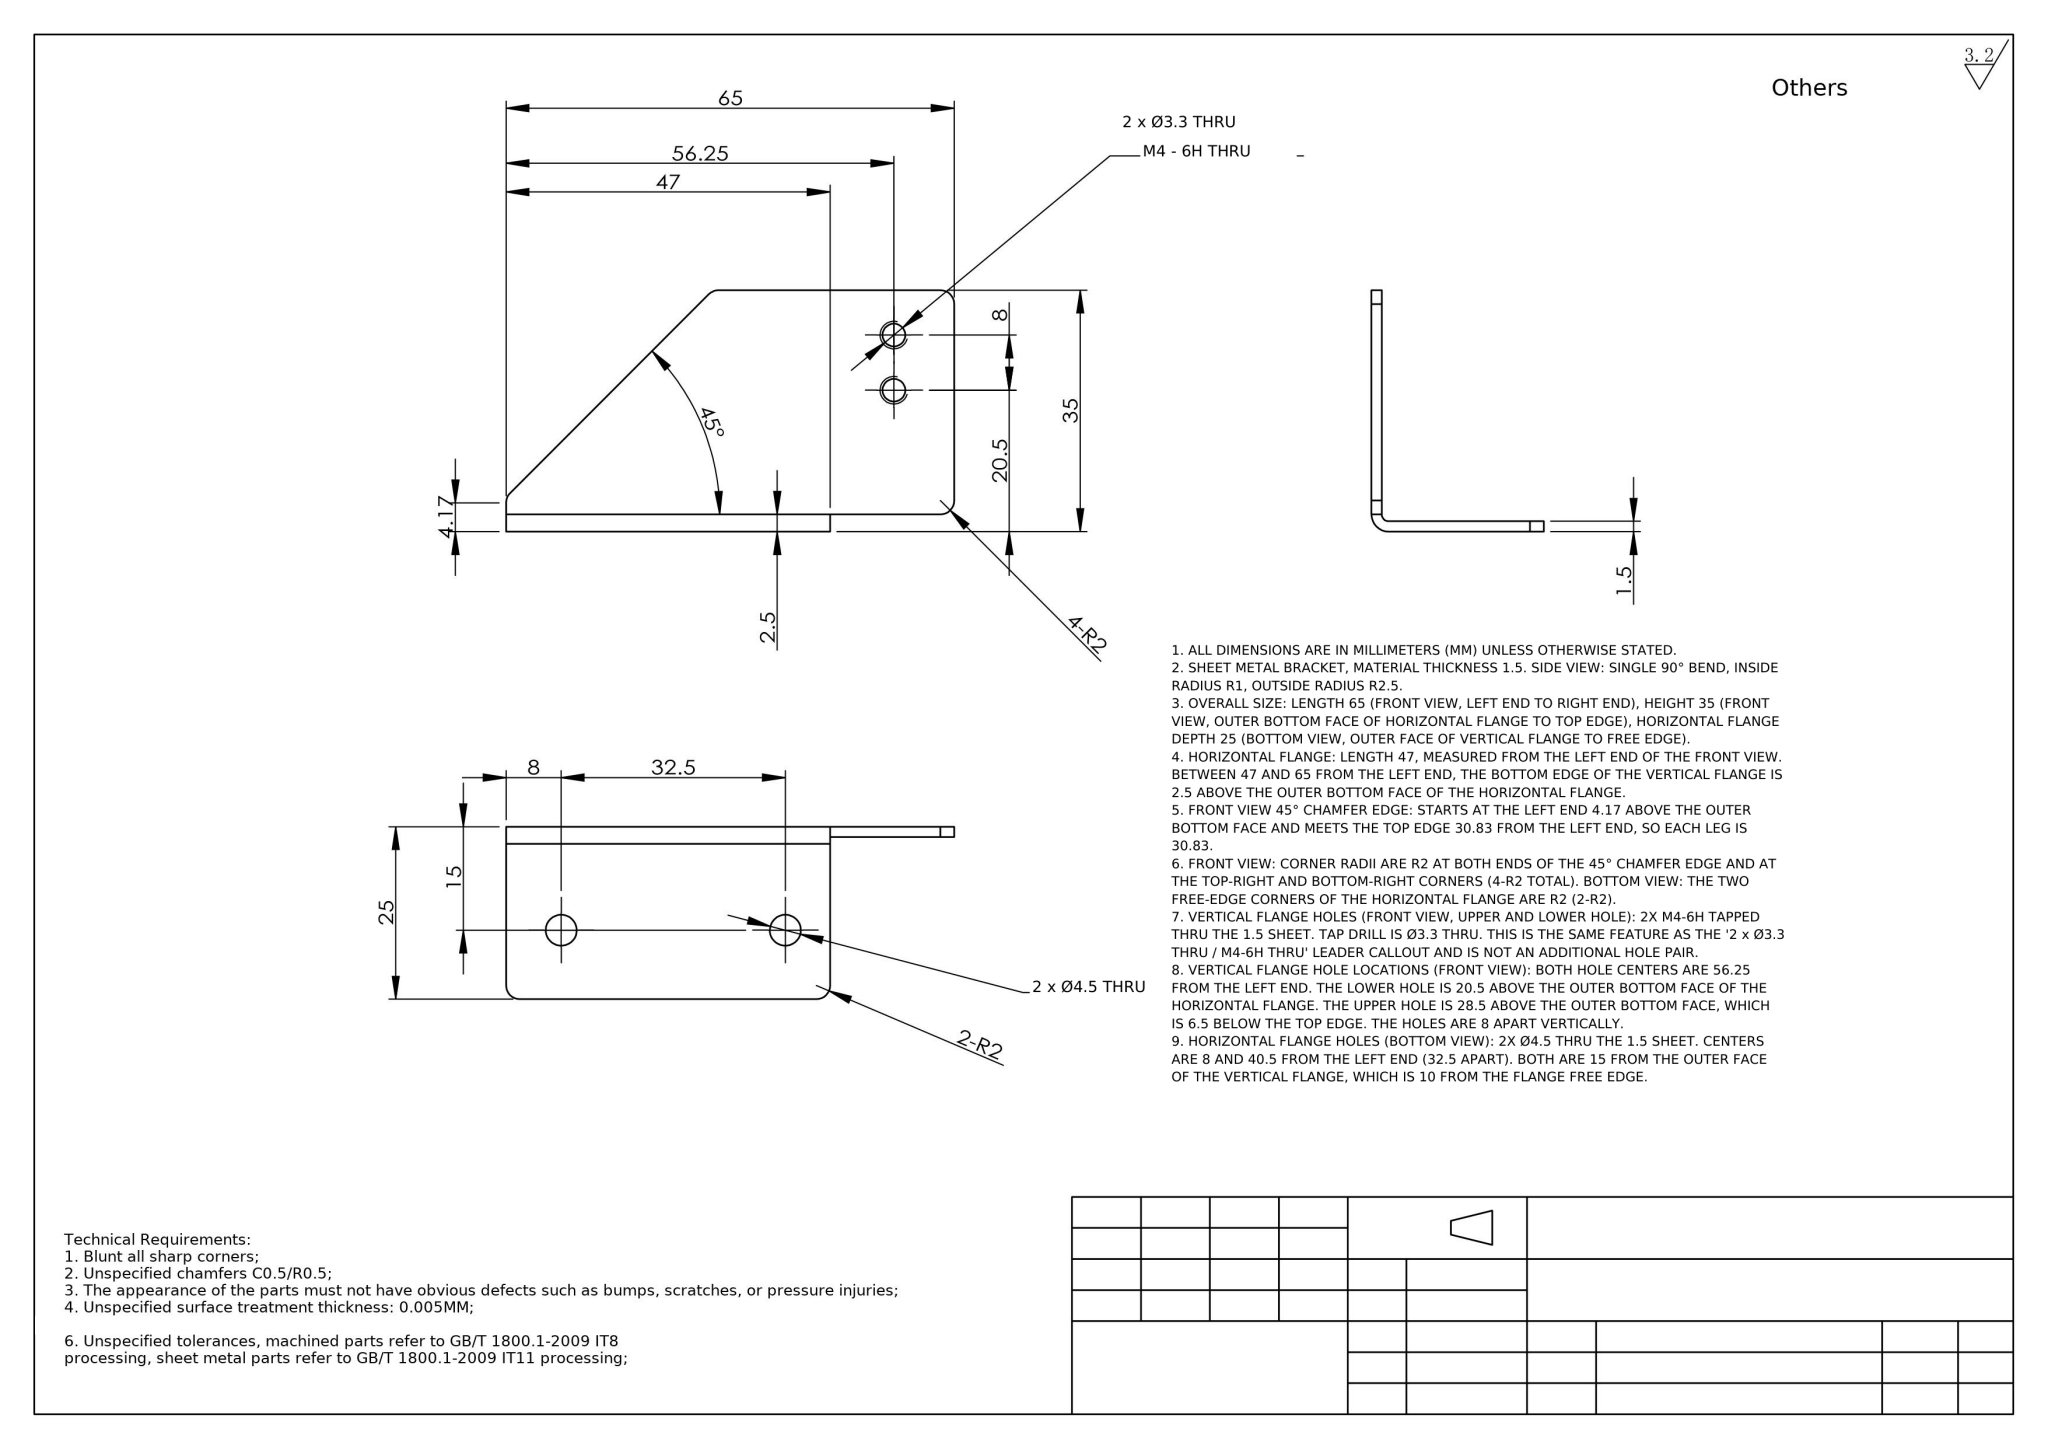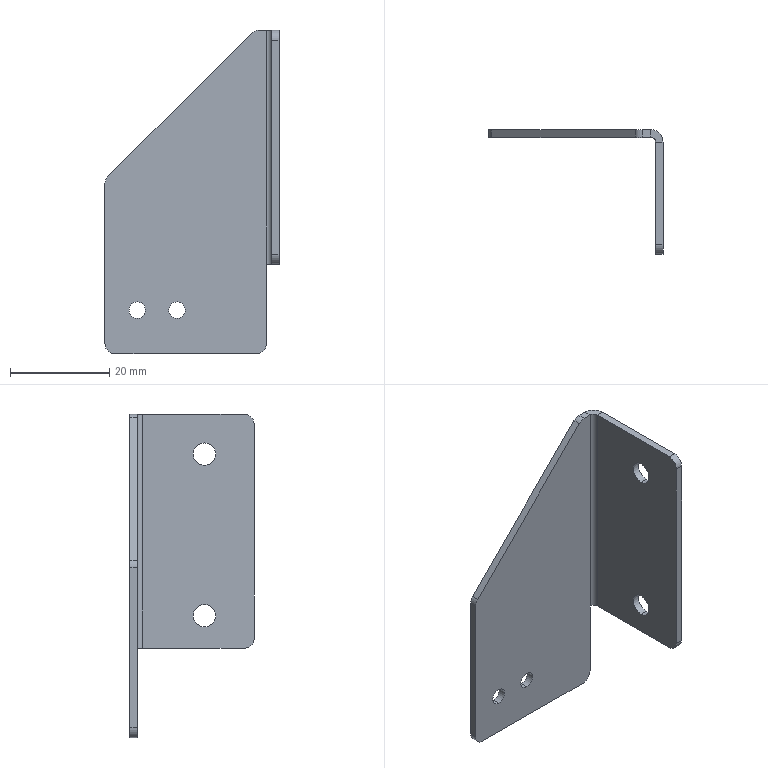Part | NX | mm | 1 solid | 29 faces | box 35 x 25 x 65 mm | volume 4195 mm3 | cylinder 16 | plane 13 | commonest cylinder face diameters 4 x6 3.3 x4 4.5 x4 5 x1 2 x1
STEP:
#1=COLOUR_RGB('',0.7529,0.7529,0.7529);
#2=FILL_AREA_STYLE_COLOUR('',#1);
#3=FILL_AREA_STYLE('',(#2));
#4=SURFACE_STYLE_FILL_AREA(#3);
#5=SURFACE_SIDE_STYLE('',(#4));
#6=SURFACE_STYLE_USAGE(.BOTH.,#5);
#7=PRESENTATION_STYLE_ASSIGNMENT((#6));
#8=CARTESIAN_POINT('',(-28.5,-1.5,7.1));
#9=VERTEX_POINT('',#8);
#10=CARTESIAN_POINT('',(-28.5,-1.5,10.4));
#11=VERTEX_POINT('',#10);
#12=CARTESIAN_POINT('',(-28.5,-1.5,8.75));
#13=DIRECTION('',(-0.,1.,0.));
#14=DIRECTION('',(-1.,-0.,0.));
#15=AXIS2_PLACEMENT_3D('',#12,#13,#14);
#16=CIRCLE('',#15,1.65);
#17=EDGE_CURVE('',#9,#11,#16,.T.);
#18=ORIENTED_EDGE('',*,*,#17,.F.);
#19=CARTESIAN_POINT('',(-28.5,-0.,7.1));
#20=VERTEX_POINT('',#19);
#21=CARTESIAN_POINT('',(-28.5,-0.,7.1));
#22=DIRECTION('',(0.,1.,0.));
#23=VECTOR('',#22,1000.);
#24=LINE('',#21,#23);
#25=EDGE_CURVE('',#9,#20,#24,.T.);
#26=ORIENTED_EDGE('',*,*,#25,.T.);
#27=CARTESIAN_POINT('',(-28.5,-0.,10.4));
#28=VERTEX_POINT('',#27);
#29=CARTESIAN_POINT('',(-28.5,-0.,8.75));
#30=DIRECTION('',(0.,1.,0.));
#31=DIRECTION('',(0.,0.,1.));
#32=AXIS2_PLACEMENT_3D('',#29,#30,#31);
#33=CIRCLE('',#32,1.65);
#34=EDGE_CURVE('',#20,#28,#33,.T.);
#35=ORIENTED_EDGE('',*,*,#34,.T.);
#36=CARTESIAN_POINT('',(-28.5,-0.,10.4));
#37=DIRECTION('',(0.,1.,0.));
#38=VECTOR('',#37,1000.);
#39=LINE('',#36,#38);
#40=EDGE_CURVE('',#11,#28,#39,.T.);
#41=ORIENTED_EDGE('',*,*,#40,.F.);
#42=EDGE_LOOP('',(#18,#26,#35,#41));
#43=FACE_OUTER_BOUND('',#42,.T.);
#44=CARTESIAN_POINT('',(-28.5,-0.,8.75));
#45=DIRECTION('',(0.,1.,0.));
#46=DIRECTION('',(0.,0.,1.));
#47=AXIS2_PLACEMENT_3D('',#44,#45,#46);
#48=CYLINDRICAL_SURFACE('',#47,1.65);
#49=ADVANCED_FACE('',(#43),#48,.F.);
#50=CARTESIAN_POINT('',(-20.5,-1.5,7.1));
#51=VERTEX_POINT('',#50);
#52=CARTESIAN_POINT('',(-20.5,-1.5,10.4));
#53=VERTEX_POINT('',#52);
#54=CARTESIAN_POINT('',(-20.5,-1.5,8.75));
#55=DIRECTION('',(-0.,1.,0.));
#56=DIRECTION('',(-1.,-0.,0.));
#57=AXIS2_PLACEMENT_3D('',#54,#55,#56);
#58=CIRCLE('',#57,1.65);
#59=EDGE_CURVE('',#51,#53,#58,.T.);
#60=ORIENTED_EDGE('',*,*,#59,.F.);
#61=CARTESIAN_POINT('',(-20.5,-0.,7.1));
#62=VERTEX_POINT('',#61);
#63=CARTESIAN_POINT('',(-20.5,-0.,7.1));
#64=DIRECTION('',(0.,1.,0.));
#65=VECTOR('',#64,1000.);
#66=LINE('',#63,#65);
#67=EDGE_CURVE('',#51,#62,#66,.T.);
#68=ORIENTED_EDGE('',*,*,#67,.T.);
#69=CARTESIAN_POINT('',(-20.5,-0.,10.4));
#70=VERTEX_POINT('',#69);
#71=CARTESIAN_POINT('',(-20.5,-0.,8.75));
#72=DIRECTION('',(0.,1.,0.));
#73=DIRECTION('',(0.,0.,1.));
#74=AXIS2_PLACEMENT_3D('',#71,#72,#73);
#75=CIRCLE('',#74,1.65);
#76=EDGE_CURVE('',#62,#70,#75,.T.);
#77=ORIENTED_EDGE('',*,*,#76,.T.);
#78=CARTESIAN_POINT('',(-20.5,-0.,10.4));
#79=DIRECTION('',(0.,1.,0.));
#80=VECTOR('',#79,1000.);
#81=LINE('',#78,#80);
#82=EDGE_CURVE('',#53,#70,#81,.T.);
#83=ORIENTED_EDGE('',*,*,#82,.F.);
#84=EDGE_LOOP('',(#60,#68,#77,#83));
#85=FACE_OUTER_BOUND('',#84,.T.);
#86=CARTESIAN_POINT('',(-20.5,-0.,8.75));
#87=DIRECTION('',(0.,1.,0.));
#88=DIRECTION('',(0.,0.,1.));
#89=AXIS2_PLACEMENT_3D('',#86,#87,#88);
#90=CYLINDRICAL_SURFACE('',#89,1.65);
#91=ADVANCED_FACE('',(#85),#90,.F.);
#92=CARTESIAN_POINT('',(0.,-15.,26.75));
#93=VERTEX_POINT('',#92);
#94=CARTESIAN_POINT('',(0.,-15.,22.25));
#95=VERTEX_POINT('',#94);
#96=CARTESIAN_POINT('',(0.,-15.,24.5));
#97=DIRECTION('',(1.,0.,0.));
#98=DIRECTION('',(-0.,1.,0.));
#99=AXIS2_PLACEMENT_3D('',#96,#97,#98);
#100=CIRCLE('',#99,2.25);
#101=EDGE_CURVE('',#93,#95,#100,.T.);
#102=ORIENTED_EDGE('',*,*,#101,.T.);
#103=CARTESIAN_POINT('',(-1.5,-15.,22.25));
#104=VERTEX_POINT('',#103);
#105=CARTESIAN_POINT('',(-1.5,-15.,22.25));
#106=DIRECTION('',(-1.,0.,0.));
#107=VECTOR('',#106,1000.);
#108=LINE('',#105,#107);
#109=EDGE_CURVE('',#95,#104,#108,.T.);
#110=ORIENTED_EDGE('',*,*,#109,.T.);
#111=CARTESIAN_POINT('',(-1.5,-15.,26.75));
#112=VERTEX_POINT('',#111);
#113=CARTESIAN_POINT('',(-1.5,-15.,24.5));
#114=DIRECTION('',(-1.,0.,0.));
#115=DIRECTION('',(0.,0.,1.));
#116=AXIS2_PLACEMENT_3D('',#113,#114,#115);
#117=CIRCLE('',#116,2.25);
#118=EDGE_CURVE('',#104,#112,#117,.T.);
#119=ORIENTED_EDGE('',*,*,#118,.T.);
#120=CARTESIAN_POINT('',(-1.5,-15.,26.75));
#121=DIRECTION('',(-1.,0.,0.));
#122=VECTOR('',#121,1000.);
#123=LINE('',#120,#122);
#124=EDGE_CURVE('',#93,#112,#123,.T.);
#125=ORIENTED_EDGE('',*,*,#124,.F.);
#126=EDGE_LOOP('',(#102,#110,#119,#125));
#127=FACE_OUTER_BOUND('',#126,.T.);
#128=CARTESIAN_POINT('',(-1.5,-15.,24.5));
#129=DIRECTION('',(-1.,0.,0.));
#130=DIRECTION('',(0.,0.,1.));
#131=AXIS2_PLACEMENT_3D('',#128,#129,#130);
#132=CYLINDRICAL_SURFACE('',#131,2.25);
#133=ADVANCED_FACE('',(#127),#132,.F.);
#134=CARTESIAN_POINT('',(0.,-15.,59.25));
#135=VERTEX_POINT('',#134);
#136=CARTESIAN_POINT('',(0.,-15.,54.75));
#137=VERTEX_POINT('',#136);
#138=CARTESIAN_POINT('',(0.,-15.,57.));
#139=DIRECTION('',(1.,0.,0.));
#140=DIRECTION('',(-0.,1.,0.));
#141=AXIS2_PLACEMENT_3D('',#138,#139,#140);
#142=CIRCLE('',#141,2.25);
#143=EDGE_CURVE('',#135,#137,#142,.T.);
#144=ORIENTED_EDGE('',*,*,#143,.T.);
#145=CARTESIAN_POINT('',(-1.5,-15.,54.75));
#146=VERTEX_POINT('',#145);
#147=CARTESIAN_POINT('',(-1.5,-15.,54.75));
#148=DIRECTION('',(-1.,0.,0.));
#149=VECTOR('',#148,1000.);
#150=LINE('',#147,#149);
#151=EDGE_CURVE('',#137,#146,#150,.T.);
#152=ORIENTED_EDGE('',*,*,#151,.T.);
#153=CARTESIAN_POINT('',(-1.5,-15.,59.25));
#154=VERTEX_POINT('',#153);
#155=CARTESIAN_POINT('',(-1.5,-15.,57.));
#156=DIRECTION('',(-1.,0.,0.));
#157=DIRECTION('',(0.,0.,1.));
#158=AXIS2_PLACEMENT_3D('',#155,#156,#157);
#159=CIRCLE('',#158,2.25);
#160=EDGE_CURVE('',#146,#154,#159,.T.);
#161=ORIENTED_EDGE('',*,*,#160,.T.);
#162=CARTESIAN_POINT('',(-1.5,-15.,59.25));
#163=DIRECTION('',(-1.,0.,0.));
#164=VECTOR('',#163,1000.);
#165=LINE('',#162,#164);
#166=EDGE_CURVE('',#135,#154,#165,.T.);
#167=ORIENTED_EDGE('',*,*,#166,.F.);
#168=EDGE_LOOP('',(#144,#152,#161,#167));
#169=FACE_OUTER_BOUND('',#168,.T.);
#170=CARTESIAN_POINT('',(-1.5,-15.,57.));
#171=DIRECTION('',(-1.,0.,0.));
#172=DIRECTION('',(0.,0.,1.));
#173=AXIS2_PLACEMENT_3D('',#170,#171,#172);
#174=CYLINDRICAL_SURFACE('',#173,2.25);
#175=ADVANCED_FACE('',(#169),#174,.F.);
#176=CARTESIAN_POINT('',(0.,-2.5,65.));
#177=VERTEX_POINT('',#176);
#178=CARTESIAN_POINT('',(-1.5,-2.5,65.));
#179=VERTEX_POINT('',#178);
#180=CARTESIAN_POINT('',(0.,-2.5,65.));
#181=DIRECTION('',(-1.,0.,0.));
#182=VECTOR('',#181,1000.);
#183=LINE('',#180,#182);
#184=EDGE_CURVE('',#177,#179,#183,.T.);
#185=ORIENTED_EDGE('',*,*,#184,.F.);
#186=CARTESIAN_POINT('',(-2.5,-0.,65.));
#187=VERTEX_POINT('',#186);
#188=CARTESIAN_POINT('',(-2.5,-2.5,65.));
#189=DIRECTION('',(0.,0.,-1.));
#190=DIRECTION('',(-1.,0.,0.));
#191=AXIS2_PLACEMENT_3D('',#188,#189,#190);
#192=CIRCLE('',#191,2.5);
#193=EDGE_CURVE('',#187,#177,#192,.T.);
#194=ORIENTED_EDGE('',*,*,#193,.F.);
#195=CARTESIAN_POINT('',(-2.5,-1.5,65.));
#196=VERTEX_POINT('',#195);
#197=CARTESIAN_POINT('',(-2.5,-1.5,65.));
#198=DIRECTION('',(-0.,1.,0.));
#199=VECTOR('',#198,1000.);
#200=LINE('',#197,#199);
#201=EDGE_CURVE('',#196,#187,#200,.T.);
#202=ORIENTED_EDGE('',*,*,#201,.F.);
#203=CARTESIAN_POINT('',(-2.5,-2.5,65.));
#204=DIRECTION('',(0.,0.,-1.));
#205=DIRECTION('',(1.,-0.,0.));
#206=AXIS2_PLACEMENT_3D('',#203,#204,#205);
#207=CIRCLE('',#206,1.);
#208=EDGE_CURVE('',#196,#179,#207,.T.);
#209=ORIENTED_EDGE('',*,*,#208,.T.);
#210=EDGE_LOOP('',(#185,#194,#202,#209));
#211=FACE_OUTER_BOUND('',#210,.T.);
#212=CARTESIAN_POINT('',(0.,-2.5,65.));
#213=DIRECTION('',(0.,0.,1.));
#214=DIRECTION('',(1.,0.,0.));
#215=AXIS2_PLACEMENT_3D('',#212,#213,#214);
#216=PLANE('',#215);
#217=ADVANCED_FACE('',(#211),#216,.T.);
#218=CARTESIAN_POINT('',(-1.5,-23.,65.));
#219=VERTEX_POINT('',#218);
#220=CARTESIAN_POINT('',(-1.5,-0.,65.));
#221=DIRECTION('',(0.,-1.,0.));
#222=VECTOR('',#221,1000.);
#223=LINE('',#220,#222);
#224=EDGE_CURVE('',#179,#219,#223,.T.);
#225=ORIENTED_EDGE('',*,*,#224,.T.);
#226=CARTESIAN_POINT('',(0.,-23.,65.));
#227=VERTEX_POINT('',#226);
#228=CARTESIAN_POINT('',(-2.5,-23.,65.));
#229=DIRECTION('',(1.,0.,0.));
#230=VECTOR('',#229,1000.);
#231=LINE('',#228,#230);
#232=EDGE_CURVE('',#219,#227,#231,.T.);
#233=ORIENTED_EDGE('',*,*,#232,.T.);
#234=CARTESIAN_POINT('',(0.,0.,65.));
#235=DIRECTION('',(0.,-1.,0.));
#236=VECTOR('',#235,1000.);
#237=LINE('',#234,#236);
#238=EDGE_CURVE('',#177,#227,#237,.T.);
#239=ORIENTED_EDGE('',*,*,#238,.F.);
#240=ORIENTED_EDGE('',*,*,#184,.T.);
#241=EDGE_LOOP('',(#225,#233,#239,#240));
#242=FACE_OUTER_BOUND('',#241,.T.);
#243=CARTESIAN_POINT('',(-2.5,-1.5,65.));
#244=DIRECTION('',(0.,0.,1.));
#245=DIRECTION('',(1.,0.,0.));
#246=AXIS2_PLACEMENT_3D('',#243,#244,#245);
#247=PLANE('',#246);
#248=ADVANCED_FACE('',(#242),#247,.T.);
#249=CARTESIAN_POINT('',(-33.,-1.5,0.));
#250=VERTEX_POINT('',#249);
#251=CARTESIAN_POINT('',(-4.5,-1.5,0.));
#252=VERTEX_POINT('',#251);
#253=CARTESIAN_POINT('',(0.,-1.5,0.));
#254=DIRECTION('',(1.,0.,0.));
#255=VECTOR('',#254,1000.);
#256=LINE('',#253,#255);
#257=EDGE_CURVE('',#250,#252,#256,.T.);
#258=ORIENTED_EDGE('',*,*,#257,.F.);
#259=CARTESIAN_POINT('',(-33.,-0.,0.));
#260=VERTEX_POINT('',#259);
#261=CARTESIAN_POINT('',(-33.,-2.5,0.));
#262=DIRECTION('',(0.,1.,0.));
#263=VECTOR('',#262,1000.);
#264=LINE('',#261,#263);
#265=EDGE_CURVE('',#250,#260,#264,.T.);
#266=ORIENTED_EDGE('',*,*,#265,.T.);
#267=CARTESIAN_POINT('',(-4.5,-0.,0.));
#268=VERTEX_POINT('',#267);
#269=CARTESIAN_POINT('',(0.,0.,0.));
#270=DIRECTION('',(1.,0.,0.));
#271=VECTOR('',#270,1000.);
#272=LINE('',#269,#271);
#273=EDGE_CURVE('',#260,#268,#272,.T.);
#274=ORIENTED_EDGE('',*,*,#273,.T.);
#275=CARTESIAN_POINT('',(-4.5,-1.5,0.));
#276=DIRECTION('',(0.,-1.,0.));
#277=VECTOR('',#276,1000.);
#278=LINE('',#275,#277);
#279=EDGE_CURVE('',#268,#252,#278,.T.);
#280=ORIENTED_EDGE('',*,*,#279,.T.);
#281=EDGE_LOOP('',(#258,#266,#274,#280));
#282=FACE_OUTER_BOUND('',#281,.T.);
#283=CARTESIAN_POINT('',(-1.5,-2.5,0.));
#284=DIRECTION('',(0.,0.,-1.));
#285=DIRECTION('',(-1.,0.,0.));
#286=AXIS2_PLACEMENT_3D('',#283,#284,#285);
#287=PLANE('',#286);
#288=ADVANCED_FACE('',(#282),#287,.T.);
#289=CARTESIAN_POINT('',(-1.5,-15.,24.5));
#290=DIRECTION('',(-1.,0.,0.));
#291=DIRECTION('',(0.,0.,1.));
#292=AXIS2_PLACEMENT_3D('',#289,#290,#291);
#293=CIRCLE('',#292,2.25);
#294=EDGE_CURVE('',#112,#104,#293,.T.);
#295=ORIENTED_EDGE('',*,*,#294,.F.);
#296=ORIENTED_EDGE('',*,*,#118,.F.);
#297=EDGE_LOOP('',(#295,#296));
#298=FACE_BOUND('',#297,.T.);
#299=CARTESIAN_POINT('',(-1.5,-15.,57.));
#300=DIRECTION('',(-1.,0.,0.));
#301=DIRECTION('',(0.,0.,1.));
#302=AXIS2_PLACEMENT_3D('',#299,#300,#301);
#303=CIRCLE('',#302,2.25);
#304=EDGE_CURVE('',#154,#146,#303,.T.);
#305=ORIENTED_EDGE('',*,*,#304,.F.);
#306=ORIENTED_EDGE('',*,*,#160,.F.);
#307=EDGE_LOOP('',(#305,#306));
#308=FACE_BOUND('',#307,.T.);
#309=CARTESIAN_POINT('',(-1.5,-2.5,18.));
#310=VERTEX_POINT('',#309);
#311=CARTESIAN_POINT('',(-1.5,-23.,18.));
#312=VERTEX_POINT('',#311);
#313=CARTESIAN_POINT('',(-1.5,-0.,18.));
#314=DIRECTION('',(0.,-1.,0.));
#315=VECTOR('',#314,1000.);
#316=LINE('',#313,#315);
#317=EDGE_CURVE('',#310,#312,#316,.T.);
#318=ORIENTED_EDGE('',*,*,#317,.T.);
#319=CARTESIAN_POINT('',(-1.5,-25.,20.));
#320=VERTEX_POINT('',#319);
#321=CARTESIAN_POINT('',(-1.5,-23.,20.));
#322=DIRECTION('',(-1.,-0.,0.));
#323=DIRECTION('',(-0.,1.,0.));
#324=AXIS2_PLACEMENT_3D('',#321,#322,#323);
#325=CIRCLE('',#324,2.);
#326=EDGE_CURVE('',#312,#320,#325,.T.);
#327=ORIENTED_EDGE('',*,*,#326,.T.);
#328=CARTESIAN_POINT('',(-1.5,-25.,63.));
#329=VERTEX_POINT('',#328);
#330=CARTESIAN_POINT('',(-1.5,-25.,65.));
#331=DIRECTION('',(0.,0.,-1.));
#332=VECTOR('',#331,1000.);
#333=LINE('',#330,#332);
#334=EDGE_CURVE('',#329,#320,#333,.T.);
#335=ORIENTED_EDGE('',*,*,#334,.F.);
#336=CARTESIAN_POINT('',(-1.5,-23.,63.));
#337=DIRECTION('',(-1.,-0.,0.));
#338=DIRECTION('',(-0.,1.,0.));
#339=AXIS2_PLACEMENT_3D('',#336,#337,#338);
#340=CIRCLE('',#339,2.);
#341=EDGE_CURVE('',#329,#219,#340,.T.);
#342=ORIENTED_EDGE('',*,*,#341,.T.);
#343=ORIENTED_EDGE('',*,*,#224,.F.);
#344=CARTESIAN_POINT('',(-1.5,-2.5,65.));
#345=DIRECTION('',(0.,0.,-1.));
#346=VECTOR('',#345,1000.);
#347=LINE('',#344,#346);
#348=EDGE_CURVE('',#179,#310,#347,.T.);
#349=ORIENTED_EDGE('',*,*,#348,.T.);
#350=EDGE_LOOP('',(#318,#327,#335,#342,#343,#349));
#351=FACE_OUTER_BOUND('',#350,.T.);
#352=CARTESIAN_POINT('',(-1.5,-0.,65.));
#353=DIRECTION('',(1.,0.,0.));
#354=DIRECTION('',(-0.,1.,0.));
#355=AXIS2_PLACEMENT_3D('',#352,#353,#354);
#356=PLANE('',#355);
#357=ADVANCED_FACE('',(#298,#308,#351),#356,.F.);
#358=ORIENTED_EDGE('',*,*,#334,.T.);
#359=CARTESIAN_POINT('',(0.,-25.,20.));
#360=VERTEX_POINT('',#359);
#361=CARTESIAN_POINT('',(0.,-25.,20.));
#362=DIRECTION('',(1.,0.,-0.));
#363=VECTOR('',#362,1000.);
#364=LINE('',#361,#363);
#365=EDGE_CURVE('',#320,#360,#364,.T.);
#366=ORIENTED_EDGE('',*,*,#365,.T.);
#367=CARTESIAN_POINT('',(0.,-25.,63.));
#368=VERTEX_POINT('',#367);
#369=CARTESIAN_POINT('',(0.,-25.,65.));
#370=DIRECTION('',(0.,0.,-1.));
#371=VECTOR('',#370,1000.);
#372=LINE('',#369,#371);
#373=EDGE_CURVE('',#368,#360,#372,.T.);
#374=ORIENTED_EDGE('',*,*,#373,.F.);
#375=CARTESIAN_POINT('',(0.,-25.,63.));
#376=DIRECTION('',(-1.,0.,0.));
#377=VECTOR('',#376,1000.);
#378=LINE('',#375,#377);
#379=EDGE_CURVE('',#368,#329,#378,.T.);
#380=ORIENTED_EDGE('',*,*,#379,.T.);
#381=EDGE_LOOP('',(#358,#366,#374,#380));
#382=FACE_OUTER_BOUND('',#381,.T.);
#383=CARTESIAN_POINT('',(0.,-25.,65.));
#384=DIRECTION('',(0.,-1.,0.));
#385=DIRECTION('',(0.,0.,-1.));
#386=AXIS2_PLACEMENT_3D('',#383,#384,#385);
#387=PLANE('',#386);
#388=ADVANCED_FACE('',(#382),#387,.T.);
#389=ORIENTED_EDGE('',*,*,#101,.F.);
#390=CARTESIAN_POINT('',(0.,-15.,24.5));
#391=DIRECTION('',(1.,0.,0.));
#392=DIRECTION('',(-0.,1.,0.));
#393=AXIS2_PLACEMENT_3D('',#390,#391,#392);
#394=CIRCLE('',#393,2.25);
#395=EDGE_CURVE('',#95,#93,#394,.T.);
#396=ORIENTED_EDGE('',*,*,#395,.F.);
#397=EDGE_LOOP('',(#389,#396));
#398=FACE_BOUND('',#397,.T.);
#399=ORIENTED_EDGE('',*,*,#143,.F.);
#400=CARTESIAN_POINT('',(0.,-15.,57.));
#401=DIRECTION('',(1.,0.,0.));
#402=DIRECTION('',(-0.,1.,0.));
#403=AXIS2_PLACEMENT_3D('',#400,#401,#402);
#404=CIRCLE('',#403,2.25);
#405=EDGE_CURVE('',#137,#135,#404,.T.);
#406=ORIENTED_EDGE('',*,*,#405,.F.);
#407=EDGE_LOOP('',(#399,#406));
#408=FACE_BOUND('',#407,.T.);
#409=ORIENTED_EDGE('',*,*,#373,.T.);
#410=CARTESIAN_POINT('',(0.,-23.,18.));
#411=VERTEX_POINT('',#410);
#412=CARTESIAN_POINT('',(0.,-23.,20.));
#413=DIRECTION('',(1.,0.,0.));
#414=DIRECTION('',(-0.,1.,0.));
#415=AXIS2_PLACEMENT_3D('',#412,#413,#414);
#416=CIRCLE('',#415,2.);
#417=EDGE_CURVE('',#360,#411,#416,.T.);
#418=ORIENTED_EDGE('',*,*,#417,.T.);
#419=CARTESIAN_POINT('',(0.,-2.5,18.));
#420=VERTEX_POINT('',#419);
#421=CARTESIAN_POINT('',(0.,0.,18.));
#422=DIRECTION('',(0.,-1.,0.));
#423=VECTOR('',#422,1000.);
#424=LINE('',#421,#423);
#425=EDGE_CURVE('',#420,#411,#424,.T.);
#426=ORIENTED_EDGE('',*,*,#425,.F.);
#427=CARTESIAN_POINT('',(0.,-2.5,65.));
#428=DIRECTION('',(0.,0.,-1.));
#429=VECTOR('',#428,1000.);
#430=LINE('',#427,#429);
#431=EDGE_CURVE('',#177,#420,#430,.T.);
#432=ORIENTED_EDGE('',*,*,#431,.F.);
#433=ORIENTED_EDGE('',*,*,#238,.T.);
#434=CARTESIAN_POINT('',(0.,-23.,63.));
#435=DIRECTION('',(1.,0.,0.));
#436=DIRECTION('',(-0.,1.,0.));
#437=AXIS2_PLACEMENT_3D('',#434,#435,#436);
#438=CIRCLE('',#437,2.);
#439=EDGE_CURVE('',#227,#368,#438,.T.);
#440=ORIENTED_EDGE('',*,*,#439,.T.);
#441=EDGE_LOOP('',(#409,#418,#426,#432,#433,#440));
#442=FACE_OUTER_BOUND('',#441,.T.);
#443=CARTESIAN_POINT('',(0.,0.,65.));
#444=DIRECTION('',(1.,0.,0.));
#445=DIRECTION('',(-0.,1.,0.));
#446=AXIS2_PLACEMENT_3D('',#443,#444,#445);
#447=PLANE('',#446);
#448=ADVANCED_FACE('',(#398,#408,#442),#447,.T.);
#449=CARTESIAN_POINT('',(-2.5,-0.,18.));
#450=VERTEX_POINT('',#449);
#451=CARTESIAN_POINT('',(-2.5,-2.5,18.));
#452=DIRECTION('',(-0.,-0.,-1.));
#453=DIRECTION('',(1.,0.,0.));
#454=AXIS2_PLACEMENT_3D('',#451,#452,#453);
#455=CIRCLE('',#454,2.5);
#456=EDGE_CURVE('',#450,#420,#455,.T.);
#457=ORIENTED_EDGE('',*,*,#456,.F.);
#458=CARTESIAN_POINT('',(-2.5,-0.,65.));
#459=DIRECTION('',(0.,0.,-1.));
#460=VECTOR('',#459,1000.);
#461=LINE('',#458,#460);
#462=EDGE_CURVE('',#187,#450,#461,.T.);
#463=ORIENTED_EDGE('',*,*,#462,.F.);
#464=ORIENTED_EDGE('',*,*,#193,.T.);
#465=ORIENTED_EDGE('',*,*,#431,.T.);
#466=EDGE_LOOP('',(#457,#463,#464,#465));
#467=FACE_OUTER_BOUND('',#466,.T.);
#468=CARTESIAN_POINT('',(-2.5,-2.5,65.));
#469=DIRECTION('',(0.,0.,-1.));
#470=DIRECTION('',(-1.,0.,0.));
#471=AXIS2_PLACEMENT_3D('',#468,#469,#470);
#472=CYLINDRICAL_SURFACE('',#471,2.5);
#473=ADVANCED_FACE('',(#467),#472,.T.);
#474=CARTESIAN_POINT('',(-28.5,-0.,8.75));
#475=DIRECTION('',(0.,1.,0.));
#476=DIRECTION('',(0.,0.,1.));
#477=AXIS2_PLACEMENT_3D('',#474,#475,#476);
#478=CIRCLE('',#477,1.65);
#479=EDGE_CURVE('',#28,#20,#478,.T.);
#480=ORIENTED_EDGE('',*,*,#479,.F.);
#481=ORIENTED_EDGE('',*,*,#34,.F.);
#482=EDGE_LOOP('',(#480,#481));
#483=FACE_BOUND('',#482,.T.);
#484=CARTESIAN_POINT('',(-20.5,-0.,8.75));
#485=DIRECTION('',(0.,1.,0.));
#486=DIRECTION('',(0.,0.,1.));
#487=AXIS2_PLACEMENT_3D('',#484,#485,#486);
#488=CIRCLE('',#487,1.65);
#489=EDGE_CURVE('',#70,#62,#488,.T.);
#490=ORIENTED_EDGE('',*,*,#489,.F.);
#491=ORIENTED_EDGE('',*,*,#76,.F.);
#492=EDGE_LOOP('',(#490,#491));
#493=FACE_BOUND('',#492,.T.);
#494=CARTESIAN_POINT('',(-35.,-0.,34.172));
#495=VERTEX_POINT('',#494);
#496=CARTESIAN_POINT('',(-35.,-0.,2.));
#497=VERTEX_POINT('',#496);
#498=CARTESIAN_POINT('',(-35.,-0.,65.));
#499=DIRECTION('',(0.,0.,-1.));
#500=VECTOR('',#499,1000.);
#501=LINE('',#498,#500);
#502=EDGE_CURVE('',#495,#497,#501,.T.);
#503=ORIENTED_EDGE('',*,*,#502,.F.);
#504=CARTESIAN_POINT('',(-34.414,-0.,35.586));
#505=VERTEX_POINT('',#504);
#506=CARTESIAN_POINT('',(-33.,-0.,34.172));
#507=DIRECTION('',(-0.,1.,0.));
#508=DIRECTION('',(-1.,-0.,0.));
#509=AXIS2_PLACEMENT_3D('',#506,#507,#508);
#510=CIRCLE('',#509,2.);
#511=EDGE_CURVE('',#495,#505,#510,.T.);
#512=ORIENTED_EDGE('',*,*,#511,.T.);
#513=CARTESIAN_POINT('',(-5.586,-0.,64.414));
#514=VERTEX_POINT('',#513);
#515=CARTESIAN_POINT('',(-2.5,-0.,67.5));
#516=DIRECTION('',(0.7071,0.,0.7071));
#517=VECTOR('',#516,1000.);
#518=LINE('',#515,#517);
#519=EDGE_CURVE('',#505,#514,#518,.T.);
#520=ORIENTED_EDGE('',*,*,#519,.T.);
#521=CARTESIAN_POINT('',(-4.172,-0.,65.));
#522=VERTEX_POINT('',#521);
#523=CARTESIAN_POINT('',(-4.172,-0.,63.));
#524=DIRECTION('',(-0.,1.,0.));
#525=DIRECTION('',(-1.,-0.,0.));
#526=AXIS2_PLACEMENT_3D('',#523,#524,#525);
#527=CIRCLE('',#526,2.);
#528=EDGE_CURVE('',#514,#522,#527,.T.);
#529=ORIENTED_EDGE('',*,*,#528,.T.);
#530=CARTESIAN_POINT('',(0.,0.,65.));
#531=DIRECTION('',(1.,0.,0.));
#532=VECTOR('',#531,1000.);
#533=LINE('',#530,#532);
#534=EDGE_CURVE('',#522,#187,#533,.T.);
#535=ORIENTED_EDGE('',*,*,#534,.T.);
#536=ORIENTED_EDGE('',*,*,#462,.T.);
#537=CARTESIAN_POINT('',(-2.5,-0.,2.));
#538=VERTEX_POINT('',#537);
#539=CARTESIAN_POINT('',(-2.5,-0.,0.));
#540=DIRECTION('',(0.,0.,1.));
#541=VECTOR('',#540,1000.);
#542=LINE('',#539,#541);
#543=EDGE_CURVE('',#538,#450,#542,.T.);
#544=ORIENTED_EDGE('',*,*,#543,.F.);
#545=CARTESIAN_POINT('',(-4.5,-0.,2.));
#546=DIRECTION('',(-0.,1.,0.));
#547=DIRECTION('',(-1.,-0.,0.));
#548=AXIS2_PLACEMENT_3D('',#545,#546,#547);
#549=CIRCLE('',#548,2.);
#550=EDGE_CURVE('',#538,#268,#549,.T.);
#551=ORIENTED_EDGE('',*,*,#550,.T.);
#552=ORIENTED_EDGE('',*,*,#273,.F.);
#553=CARTESIAN_POINT('',(-33.,-0.,2.));
#554=DIRECTION('',(-0.,1.,0.));
#555=DIRECTION('',(-1.,-0.,0.));
#556=AXIS2_PLACEMENT_3D('',#553,#554,#555);
#557=CIRCLE('',#556,2.);
#558=EDGE_CURVE('',#260,#497,#557,.T.);
#559=ORIENTED_EDGE('',*,*,#558,.T.);
#560=EDGE_LOOP('',(#503,#512,#520,#529,#535,#536,#544,#551,#552,#559));
#561=FACE_OUTER_BOUND('',#560,.T.);
#562=CARTESIAN_POINT('',(0.,0.,65.));
#563=DIRECTION('',(-0.,1.,0.));
#564=DIRECTION('',(-1.,-0.,0.));
#565=AXIS2_PLACEMENT_3D('',#562,#563,#564);
#566=PLANE('',#565);
#567=ADVANCED_FACE('',(#483,#493,#561),#566,.T.);
#568=CARTESIAN_POINT('',(-35.,-1.5,34.172));
#569=VERTEX_POINT('',#568);
#570=CARTESIAN_POINT('',(-35.,-1.5,2.));
#571=VERTEX_POINT('',#570);
#572=CARTESIAN_POINT('',(-35.,-1.5,65.));
#573=DIRECTION('',(0.,0.,-1.));
#574=VECTOR('',#573,1000.);
#575=LINE('',#572,#574);
#576=EDGE_CURVE('',#569,#571,#575,.T.);
#577=ORIENTED_EDGE('',*,*,#576,.F.);
#578=CARTESIAN_POINT('',(-35.,-1.5,34.172));
#579=DIRECTION('',(0.,1.,0.));
#580=VECTOR('',#579,1000.);
#581=LINE('',#578,#580);
#582=EDGE_CURVE('',#569,#495,#581,.T.);
#583=ORIENTED_EDGE('',*,*,#582,.T.);
#584=ORIENTED_EDGE('',*,*,#502,.T.);
#585=CARTESIAN_POINT('',(-35.,-1.5,2.));
#586=DIRECTION('',(0.,-1.,0.));
#587=VECTOR('',#586,1000.);
#588=LINE('',#585,#587);
#589=EDGE_CURVE('',#497,#571,#588,.T.);
#590=ORIENTED_EDGE('',*,*,#589,.T.);
#591=EDGE_LOOP('',(#577,#583,#584,#590));
#592=FACE_OUTER_BOUND('',#591,.T.);
#593=CARTESIAN_POINT('',(-35.,-1.5,65.));
#594=DIRECTION('',(-1.,0.,0.));
#595=DIRECTION('',(0.,0.,1.));
#596=AXIS2_PLACEMENT_3D('',#593,#594,#595);
#597=PLANE('',#596);
#598=ADVANCED_FACE('',(#592),#597,.T.);
#599=CARTESIAN_POINT('',(-28.5,-1.5,8.75));
#600=DIRECTION('',(-0.,1.,0.));
#601=DIRECTION('',(-1.,-0.,0.));
#602=AXIS2_PLACEMENT_3D('',#599,#600,#601);
#603=CIRCLE('',#602,1.65);
#604=EDGE_CURVE('',#11,#9,#603,.T.);
#605=ORIENTED_EDGE('',*,*,#604,.T.);
#606=ORIENTED_EDGE('',*,*,#17,.T.);
#607=EDGE_LOOP('',(#605,#606));
#608=FACE_BOUND('',#607,.T.);
#609=CARTESIAN_POINT('',(-20.5,-1.5,8.75));
#610=DIRECTION('',(-0.,1.,0.));
#611=DIRECTION('',(-1.,-0.,0.));
#612=AXIS2_PLACEMENT_3D('',#609,#610,#611);
#613=CIRCLE('',#612,1.65);
#614=EDGE_CURVE('',#53,#51,#613,.T.);
#615=ORIENTED_EDGE('',*,*,#614,.T.);
#616=ORIENTED_EDGE('',*,*,#59,.T.);
#617=EDGE_LOOP('',(#615,#616));
#618=FACE_BOUND('',#617,.T.);
#619=CARTESIAN_POINT('',(-5.586,-1.5,64.414));
#620=VERTEX_POINT('',#619);
#621=CARTESIAN_POINT('',(-34.414,-1.5,35.586));
#622=VERTEX_POINT('',#621);
#623=CARTESIAN_POINT('',(-35.,-1.5,35.));
#624=DIRECTION('',(-0.7071,-0.,-0.7071));
#625=VECTOR('',#624,1000.);
#626=LINE('',#623,#625);
#627=EDGE_CURVE('',#620,#622,#626,.T.);
#628=ORIENTED_EDGE('',*,*,#627,.T.);
#629=CARTESIAN_POINT('',(-33.,-1.5,34.172));
#630=DIRECTION('',(0.,-1.,0.));
#631=DIRECTION('',(-1.,-0.,-0.));
#632=AXIS2_PLACEMENT_3D('',#629,#630,#631);
#633=CIRCLE('',#632,2.);
#634=EDGE_CURVE('',#622,#569,#633,.T.);
#635=ORIENTED_EDGE('',*,*,#634,.T.);
#636=ORIENTED_EDGE('',*,*,#576,.T.);
#637=CARTESIAN_POINT('',(-33.,-1.5,2.));
#638=DIRECTION('',(0.,-1.,0.));
#639=DIRECTION('',(-1.,-0.,0.));
#640=AXIS2_PLACEMENT_3D('',#637,#638,#639);
#641=CIRCLE('',#640,2.);
#642=EDGE_CURVE('',#571,#250,#641,.T.);
#643=ORIENTED_EDGE('',*,*,#642,.T.);
#644=ORIENTED_EDGE('',*,*,#257,.T.);
#645=CARTESIAN_POINT('',(-2.5,-1.5,2.));
#646=VERTEX_POINT('',#645);
#647=CARTESIAN_POINT('',(-4.5,-1.5,2.));
#648=DIRECTION('',(0.,-1.,0.));
#649=DIRECTION('',(-1.,-0.,0.));
#650=AXIS2_PLACEMENT_3D('',#647,#648,#649);
#651=CIRCLE('',#650,2.);
#652=EDGE_CURVE('',#252,#646,#651,.T.);
#653=ORIENTED_EDGE('',*,*,#652,.T.);
#654=CARTESIAN_POINT('',(-2.5,-1.5,18.));
#655=VERTEX_POINT('',#654);
#656=CARTESIAN_POINT('',(-2.5,-1.5,65.));
#657=DIRECTION('',(0.,0.,-1.));
#658=VECTOR('',#657,1000.);
#659=LINE('',#656,#658);
#660=EDGE_CURVE('',#655,#646,#659,.T.);
#661=ORIENTED_EDGE('',*,*,#660,.F.);
#662=CARTESIAN_POINT('',(-2.5,-1.5,65.));
#663=DIRECTION('',(0.,0.,-1.));
#664=VECTOR('',#663,1000.);
#665=LINE('',#662,#664);
#666=EDGE_CURVE('',#196,#655,#665,.T.);
#667=ORIENTED_EDGE('',*,*,#666,.F.);
#668=CARTESIAN_POINT('',(-4.172,-1.5,65.));
#669=VERTEX_POINT('',#668);
#670=CARTESIAN_POINT('',(0.,-1.5,65.));
#671=DIRECTION('',(1.,0.,0.));
#672=VECTOR('',#671,1000.);
#673=LINE('',#670,#672);
#674=EDGE_CURVE('',#669,#196,#673,.T.);
#675=ORIENTED_EDGE('',*,*,#674,.F.);
#676=CARTESIAN_POINT('',(-4.172,-1.5,63.));
#677=DIRECTION('',(0.,-1.,0.));
#678=DIRECTION('',(-1.,-0.,-0.));
#679=AXIS2_PLACEMENT_3D('',#676,#677,#678);
#680=CIRCLE('',#679,2.);
#681=EDGE_CURVE('',#669,#620,#680,.T.);
#682=ORIENTED_EDGE('',*,*,#681,.T.);
#683=EDGE_LOOP('',(#628,#635,#636,#643,#644,#653,#661,#667,#675,#682));
#684=FACE_OUTER_BOUND('',#683,.T.);
#685=CARTESIAN_POINT('',(0.,-1.5,65.));
#686=DIRECTION('',(-0.,1.,0.));
#687=DIRECTION('',(-1.,-0.,0.));
#688=AXIS2_PLACEMENT_3D('',#685,#686,#687);
#689=PLANE('',#688);
#690=ADVANCED_FACE('',(#608,#618,#684),#689,.F.);
#691=ORIENTED_EDGE('',*,*,#666,.T.);
#692=CARTESIAN_POINT('',(-2.5,-2.5,18.));
#693=DIRECTION('',(-0.,-0.,-1.));
#694=DIRECTION('',(1.,0.,0.));
#695=AXIS2_PLACEMENT_3D('',#692,#693,#694);
#696=CIRCLE('',#695,1.);
#697=EDGE_CURVE('',#655,#310,#696,.T.);
#698=ORIENTED_EDGE('',*,*,#697,.T.);
#699=ORIENTED_EDGE('',*,*,#348,.F.);
#700=ORIENTED_EDGE('',*,*,#208,.F.);
#701=EDGE_LOOP('',(#691,#698,#699,#700));
#702=FACE_OUTER_BOUND('',#701,.T.);
#703=CARTESIAN_POINT('',(-2.5,-2.5,65.));
#704=DIRECTION('',(0.,0.,-1.));
#705=DIRECTION('',(-1.,0.,0.));
#706=AXIS2_PLACEMENT_3D('',#703,#704,#705);
#707=CYLINDRICAL_SURFACE('',#706,1.);
#708=ADVANCED_FACE('',(#702),#707,.F.);
#709=ORIENTED_EDGE('',*,*,#534,.F.);
#710=CARTESIAN_POINT('',(-4.172,-1.5,65.));
#711=DIRECTION('',(0.,-1.,0.));
#712=VECTOR('',#711,1000.);
#713=LINE('',#710,#712);
#714=EDGE_CURVE('',#522,#669,#713,.T.);
#715=ORIENTED_EDGE('',*,*,#714,.T.);
#716=ORIENTED_EDGE('',*,*,#674,.T.);
#717=ORIENTED_EDGE('',*,*,#201,.T.);
#718=EDGE_LOOP('',(#709,#715,#716,#717));
#719=FACE_OUTER_BOUND('',#718,.T.);
#720=CARTESIAN_POINT('',(-2.5,-2.5,65.));
#721=DIRECTION('',(0.,0.,-1.));
#722=DIRECTION('',(-1.,0.,0.));
#723=AXIS2_PLACEMENT_3D('',#720,#721,#722);
#724=PLANE('',#723);
#725=ADVANCED_FACE('',(#719),#724,.F.);
#726=ORIENTED_EDGE('',*,*,#660,.T.);
#727=CARTESIAN_POINT('',(-2.5,-0.,2.));
#728=DIRECTION('',(-0.,1.,0.));
#729=VECTOR('',#728,1000.);
#730=LINE('',#727,#729);
#731=EDGE_CURVE('',#646,#538,#730,.T.);
#732=ORIENTED_EDGE('',*,*,#731,.T.);
#733=ORIENTED_EDGE('',*,*,#543,.T.);
#734=CARTESIAN_POINT('',(-2.5,-45.,18.));
#735=DIRECTION('',(-0.,1.,0.));
#736=VECTOR('',#735,1000.);
#737=LINE('',#734,#736);
#738=EDGE_CURVE('',#655,#450,#737,.T.);
#739=ORIENTED_EDGE('',*,*,#738,.F.);
#740=EDGE_LOOP('',(#726,#732,#733,#739));
#741=FACE_OUTER_BOUND('',#740,.T.);
#742=CARTESIAN_POINT('',(-2.5,-45.,0.));
#743=DIRECTION('',(-1.,-0.,0.));
#744=DIRECTION('',(0.,-1.,0.));
#745=AXIS2_PLACEMENT_3D('',#742,#743,#744);
#746=PLANE('',#745);
#747=ADVANCED_FACE('',(#741),#746,.F.);
#748=ORIENTED_EDGE('',*,*,#425,.T.);
#749=CARTESIAN_POINT('',(-1.5,-23.,18.));
#750=DIRECTION('',(-1.,0.,0.));
#751=VECTOR('',#750,1000.);
#752=LINE('',#749,#751);
#753=EDGE_CURVE('',#411,#312,#752,.T.);
#754=ORIENTED_EDGE('',*,*,#753,.T.);
#755=ORIENTED_EDGE('',*,*,#317,.F.);
#756=ORIENTED_EDGE('',*,*,#697,.F.);
#757=ORIENTED_EDGE('',*,*,#738,.T.);
#758=ORIENTED_EDGE('',*,*,#456,.T.);
#759=EDGE_LOOP('',(#748,#754,#755,#756,#757,#758));
#760=FACE_OUTER_BOUND('',#759,.T.);
#761=CARTESIAN_POINT('',(30.,-45.,18.));
#762=DIRECTION('',(0.,0.,1.));
#763=DIRECTION('',(1.,0.,-0.));
#764=AXIS2_PLACEMENT_3D('',#761,#762,#763);
#765=PLANE('',#764);
#766=ADVANCED_FACE('',(#760),#765,.F.);
#767=ORIENTED_EDGE('',*,*,#151,.F.);
#768=ORIENTED_EDGE('',*,*,#405,.T.);
#769=ORIENTED_EDGE('',*,*,#166,.T.);
#770=ORIENTED_EDGE('',*,*,#304,.T.);
#771=EDGE_LOOP('',(#767,#768,#769,#770));
#772=FACE_OUTER_BOUND('',#771,.T.);
#773=CARTESIAN_POINT('',(-1.5,-15.,57.));
#774=DIRECTION('',(-1.,0.,0.));
#775=DIRECTION('',(0.,0.,1.));
#776=AXIS2_PLACEMENT_3D('',#773,#774,#775);
#777=CYLINDRICAL_SURFACE('',#776,2.25);
#778=ADVANCED_FACE('',(#772),#777,.F.);
#779=ORIENTED_EDGE('',*,*,#109,.F.);
#780=ORIENTED_EDGE('',*,*,#395,.T.);
#781=ORIENTED_EDGE('',*,*,#124,.T.);
#782=ORIENTED_EDGE('',*,*,#294,.T.);
#783=EDGE_LOOP('',(#779,#780,#781,#782));
#784=FACE_OUTER_BOUND('',#783,.T.);
#785=CARTESIAN_POINT('',(-1.5,-15.,24.5));
#786=DIRECTION('',(-1.,0.,0.));
#787=DIRECTION('',(0.,0.,1.));
#788=AXIS2_PLACEMENT_3D('',#785,#786,#787);
#789=CYLINDRICAL_SURFACE('',#788,2.25);
#790=ADVANCED_FACE('',(#784),#789,.F.);
#791=ORIENTED_EDGE('',*,*,#67,.F.);
#792=ORIENTED_EDGE('',*,*,#614,.F.);
#793=ORIENTED_EDGE('',*,*,#82,.T.);
#794=ORIENTED_EDGE('',*,*,#489,.T.);
#795=EDGE_LOOP('',(#791,#792,#793,#794));
#796=FACE_OUTER_BOUND('',#795,.T.);
#797=CARTESIAN_POINT('',(-20.5,-0.,8.75));
#798=DIRECTION('',(0.,1.,0.));
#799=DIRECTION('',(0.,0.,1.));
#800=AXIS2_PLACEMENT_3D('',#797,#798,#799);
#801=CYLINDRICAL_SURFACE('',#800,1.65);
#802=ADVANCED_FACE('',(#796),#801,.F.);
#803=ORIENTED_EDGE('',*,*,#25,.F.);
#804=ORIENTED_EDGE('',*,*,#604,.F.);
#805=ORIENTED_EDGE('',*,*,#40,.T.);
#806=ORIENTED_EDGE('',*,*,#479,.T.);
#807=EDGE_LOOP('',(#803,#804,#805,#806));
#808=FACE_OUTER_BOUND('',#807,.T.);
#809=CARTESIAN_POINT('',(-28.5,-0.,8.75));
#810=DIRECTION('',(0.,1.,0.));
#811=DIRECTION('',(0.,0.,1.));
#812=AXIS2_PLACEMENT_3D('',#809,#810,#811);
#813=CYLINDRICAL_SURFACE('',#812,1.65);
#814=ADVANCED_FACE('',(#808),#813,.F.);
#815=ORIENTED_EDGE('',*,*,#519,.F.);
#816=CARTESIAN_POINT('',(-34.414,-1.5,35.586));
#817=DIRECTION('',(0.,-1.,0.));
#818=VECTOR('',#817,1000.);
#819=LINE('',#816,#818);
#820=EDGE_CURVE('',#505,#622,#819,.T.);
#821=ORIENTED_EDGE('',*,*,#820,.T.);
#822=ORIENTED_EDGE('',*,*,#627,.F.);
#823=CARTESIAN_POINT('',(-5.586,-0.,64.414));
#824=DIRECTION('',(0.,1.,0.));
#825=VECTOR('',#824,1000.);
#826=LINE('',#823,#825);
#827=EDGE_CURVE('',#620,#514,#826,.T.);
#828=ORIENTED_EDGE('',*,*,#827,.T.);
#829=EDGE_LOOP('',(#815,#821,#822,#828));
#830=FACE_OUTER_BOUND('',#829,.T.);
#831=CARTESIAN_POINT('',(-35.,-1.5,35.));
#832=DIRECTION('',(-0.7071,0.,0.7071));
#833=DIRECTION('',(0.,-1.,0.));
#834=AXIS2_PLACEMENT_3D('',#831,#832,#833);
#835=PLANE('',#834);
#836=ADVANCED_FACE('',(#830),#835,.T.);
#837=ORIENTED_EDGE('',*,*,#417,.F.);
#838=ORIENTED_EDGE('',*,*,#365,.F.);
#839=ORIENTED_EDGE('',*,*,#326,.F.);
#840=ORIENTED_EDGE('',*,*,#753,.F.);
#841=EDGE_LOOP('',(#837,#838,#839,#840));
#842=FACE_OUTER_BOUND('',#841,.T.);
#843=CARTESIAN_POINT('',(30.,-23.,20.));
#844=DIRECTION('',(1.,0.,-0.));
#845=DIRECTION('',(0.,0.,-1.));
#846=AXIS2_PLACEMENT_3D('',#843,#844,#845);
#847=CYLINDRICAL_SURFACE('',#846,2.);
#848=ADVANCED_FACE('',(#842),#847,.T.);
#849=ORIENTED_EDGE('',*,*,#439,.F.);
#850=ORIENTED_EDGE('',*,*,#232,.F.);
#851=ORIENTED_EDGE('',*,*,#341,.F.);
#852=ORIENTED_EDGE('',*,*,#379,.F.);
#853=EDGE_LOOP('',(#849,#850,#851,#852));
#854=FACE_OUTER_BOUND('',#853,.T.);
#855=CARTESIAN_POINT('',(0.,-23.,63.));
#856=DIRECTION('',(-1.,0.,0.));
#857=DIRECTION('',(0.,0.,1.));
#858=AXIS2_PLACEMENT_3D('',#855,#856,#857);
#859=CYLINDRICAL_SURFACE('',#858,2.);
#860=ADVANCED_FACE('',(#854),#859,.T.);
#861=ORIENTED_EDGE('',*,*,#634,.F.);
#862=ORIENTED_EDGE('',*,*,#820,.F.);
#863=ORIENTED_EDGE('',*,*,#511,.F.);
#864=ORIENTED_EDGE('',*,*,#582,.F.);
#865=EDGE_LOOP('',(#861,#862,#863,#864));
#866=FACE_OUTER_BOUND('',#865,.T.);
#867=CARTESIAN_POINT('',(-33.,-1.5,34.172));
#868=DIRECTION('',(0.,1.,0.));
#869=DIRECTION('',(0.,0.,1.));
#870=AXIS2_PLACEMENT_3D('',#867,#868,#869);
#871=CYLINDRICAL_SURFACE('',#870,2.);
#872=ADVANCED_FACE('',(#866),#871,.T.);
#873=ORIENTED_EDGE('',*,*,#528,.F.);
#874=ORIENTED_EDGE('',*,*,#827,.F.);
#875=ORIENTED_EDGE('',*,*,#681,.F.);
#876=ORIENTED_EDGE('',*,*,#714,.F.);
#877=EDGE_LOOP('',(#873,#874,#875,#876));
#878=FACE_OUTER_BOUND('',#877,.T.);
#879=CARTESIAN_POINT('',(-4.172,-2.5,63.));
#880=DIRECTION('',(0.,1.,0.));
#881=DIRECTION('',(0.,0.,1.));
#882=AXIS2_PLACEMENT_3D('',#879,#880,#881);
#883=CYLINDRICAL_SURFACE('',#882,2.);
#884=ADVANCED_FACE('',(#878),#883,.T.);
#885=ORIENTED_EDGE('',*,*,#642,.F.);
#886=ORIENTED_EDGE('',*,*,#589,.F.);
#887=ORIENTED_EDGE('',*,*,#558,.F.);
#888=ORIENTED_EDGE('',*,*,#265,.F.);
#889=EDGE_LOOP('',(#885,#886,#887,#888));
#890=FACE_OUTER_BOUND('',#889,.T.);
#891=CARTESIAN_POINT('',(-33.,-2.5,2.));
#892=DIRECTION('',(0.,1.,0.));
#893=DIRECTION('',(0.,0.,1.));
#894=AXIS2_PLACEMENT_3D('',#891,#892,#893);
#895=CYLINDRICAL_SURFACE('',#894,2.);
#896=ADVANCED_FACE('',(#890),#895,.T.);
#897=ORIENTED_EDGE('',*,*,#550,.F.);
#898=ORIENTED_EDGE('',*,*,#731,.F.);
#899=ORIENTED_EDGE('',*,*,#652,.F.);
#900=ORIENTED_EDGE('',*,*,#279,.F.);
#901=EDGE_LOOP('',(#897,#898,#899,#900));
#902=FACE_OUTER_BOUND('',#901,.T.);
#903=CARTESIAN_POINT('',(-4.5,-2.5,2.));
#904=DIRECTION('',(-0.,1.,0.));
#905=DIRECTION('',(-1.,-0.,0.));
#906=AXIS2_PLACEMENT_3D('',#903,#904,#905);
#907=CYLINDRICAL_SURFACE('',#906,2.);
#908=ADVANCED_FACE('',(#902),#907,.T.);
#909=CLOSED_SHELL('',(#49,#91,#133,#175,#217,#248,#288,#357,#388,#448,#473,#567,#598,#690,#708,#725,#747,#766,#778,#790,#802,#814,#836,#848,#860,#872,#884,#896,#908));
#910=MANIFOLD_SOLID_BREP('',#909);
#911=STYLED_ITEM('',(#7),#910);
#912=(LENGTH_UNIT()NAMED_UNIT(*)SI_UNIT(.MILLI.,.METRE.));
#913=UNCERTAINTY_MEASURE_WITH_UNIT(LENGTH_MEASURE(0.00001),#912,'','');
#914=(NAMED_UNIT(*)PLANE_ANGLE_UNIT()SI_UNIT($,.RADIAN.));
#915=(NAMED_UNIT(*)SI_UNIT($,.STERADIAN.)SOLID_ANGLE_UNIT());
#916=(GEOMETRIC_REPRESENTATION_CONTEXT(3)GLOBAL_UNCERTAINTY_ASSIGNED_CONTEXT((#913))GLOBAL_UNIT_ASSIGNED_CONTEXT((#912,#914,#915))REPRESENTATION_CONTEXT('',''));
#917=MECHANICAL_DESIGN_GEOMETRIC_PRESENTATION_REPRESENTATION('',(#911),#916);
#918=COLOUR_RGB('',0.7529,0.7529,0.7529);
#919=FILL_AREA_STYLE_COLOUR('',#918);
#920=FILL_AREA_STYLE('',(#919));
#921=SURFACE_STYLE_FILL_AREA(#920);
#922=SURFACE_SIDE_STYLE('',(#921));
#923=SURFACE_STYLE_USAGE(.BOTH.,#922);
#924=PRESENTATION_STYLE_ASSIGNMENT((#923));
#925=STYLED_ITEM('',(#924),#802);
#926=PRESENTATION_LAYER_ASSIGNMENT('','',(#925));
#927=COLOUR_RGB('',0.7529,0.7529,0.7529);
#928=FILL_AREA_STYLE_COLOUR('',#927);
#929=FILL_AREA_STYLE('',(#928));
#930=SURFACE_STYLE_FILL_AREA(#929);
#931=SURFACE_SIDE_STYLE('',(#930));
#932=SURFACE_STYLE_USAGE(.BOTH.,#931);
#933=PRESENTATION_STYLE_ASSIGNMENT((#932));
#934=STYLED_ITEM('',(#933),#49);
#935=PRESENTATION_LAYER_ASSIGNMENT('','',(#934));
#936=COLOUR_RGB('',0.7529,0.7529,0.7529);
#937=FILL_AREA_STYLE_COLOUR('',#936);
#938=FILL_AREA_STYLE('',(#937));
#939=SURFACE_STYLE_FILL_AREA(#938);
#940=SURFACE_SIDE_STYLE('',(#939));
#941=SURFACE_STYLE_USAGE(.BOTH.,#940);
#942=PRESENTATION_STYLE_ASSIGNMENT((#941));
#943=CARTESIAN_POINT('',(0.,0.,0.));
#944=DIRECTION('',(0.,0.,1.));
#945=DIRECTION('',(1.,0.,0.));
#946=AXIS2_PLACEMENT_3D('',#943,#944,#945);
#947=(LENGTH_UNIT()NAMED_UNIT(*)SI_UNIT(.MILLI.,.METRE.));
#948=UNCERTAINTY_MEASURE_WITH_UNIT(LENGTH_MEASURE(0.00001),#947,'','');
#949=(NAMED_UNIT(*)PLANE_ANGLE_UNIT()SI_UNIT($,.RADIAN.));
#950=(NAMED_UNIT(*)SI_UNIT($,.STERADIAN.)SOLID_ANGLE_UNIT());
#951=(GEOMETRIC_REPRESENTATION_CONTEXT(3)GLOBAL_UNCERTAINTY_ASSIGNED_CONTEXT((#948))GLOBAL_UNIT_ASSIGNED_CONTEXT((#947,#949,#950))REPRESENTATION_CONTEXT('',''));
#952=ADVANCED_BREP_SHAPE_REPRESENTATION('',(#910,#946),#951);
#953=STYLED_ITEM('',(#942),#952);
#954=PRESENTATION_LAYER_ASSIGNMENT('','',(#953));
#955=COLOUR_RGB('',0.7529,0.7529,0.7529);
#956=FILL_AREA_STYLE_COLOUR('',#955);
#957=FILL_AREA_STYLE('',(#956));
#958=SURFACE_STYLE_FILL_AREA(#957);
#959=SURFACE_SIDE_STYLE('',(#958));
#960=SURFACE_STYLE_USAGE(.BOTH.,#959);
#961=PRESENTATION_STYLE_ASSIGNMENT((#960));
#962=STYLED_ITEM('',(#961),#814);
#963=PRESENTATION_LAYER_ASSIGNMENT('','',(#962));
#964=(LENGTH_UNIT()NAMED_UNIT(*)SI_UNIT(.MILLI.,.METRE.));
#965=UNCERTAINTY_MEASURE_WITH_UNIT(LENGTH_MEASURE(0.00001),#964,'','');
#966=(NAMED_UNIT(*)PLANE_ANGLE_UNIT()SI_UNIT($,.RADIAN.));
#967=(NAMED_UNIT(*)SI_UNIT($,.STERADIAN.)SOLID_ANGLE_UNIT());
#968=(GEOMETRIC_REPRESENTATION_CONTEXT(3)GLOBAL_UNCERTAINTY_ASSIGNED_CONTEXT((#965))GLOBAL_UNIT_ASSIGNED_CONTEXT((#964,#966,#967))REPRESENTATION_CONTEXT('',''));
#969=MECHANICAL_DESIGN_GEOMETRIC_PRESENTATION_REPRESENTATION('',(#934),#968);
#970=PRESENTATION_LAYER_ASSIGNMENT('','',(#911));
#971=COLOUR_RGB('',0.7529,0.7529,0.7529);
#972=FILL_AREA_STYLE_COLOUR('',#971);
#973=FILL_AREA_STYLE('',(#972));
#974=SURFACE_STYLE_FILL_AREA(#973);
#975=SURFACE_SIDE_STYLE('',(#974));
#976=SURFACE_STYLE_USAGE(.BOTH.,#975);
#977=PRESENTATION_STYLE_ASSIGNMENT((#976));
#978=STYLED_ITEM('',(#977),#91);
#979=(LENGTH_UNIT()NAMED_UNIT(*)SI_UNIT(.MILLI.,.METRE.));
#980=UNCERTAINTY_MEASURE_WITH_UNIT(LENGTH_MEASURE(0.00001),#979,'','');
#981=(NAMED_UNIT(*)PLANE_ANGLE_UNIT()SI_UNIT($,.RADIAN.));
#982=(NAMED_UNIT(*)SI_UNIT($,.STERADIAN.)SOLID_ANGLE_UNIT());
#983=(GEOMETRIC_REPRESENTATION_CONTEXT(3)GLOBAL_UNCERTAINTY_ASSIGNED_CONTEXT((#980))GLOBAL_UNIT_ASSIGNED_CONTEXT((#979,#981,#982))REPRESENTATION_CONTEXT('',''));
#984=MECHANICAL_DESIGN_GEOMETRIC_PRESENTATION_REPRESENTATION('',(#978),#983);
#985=(LENGTH_UNIT()NAMED_UNIT(*)SI_UNIT(.MILLI.,.METRE.));
#986=UNCERTAINTY_MEASURE_WITH_UNIT(LENGTH_MEASURE(0.00001),#985,'','');
#987=(NAMED_UNIT(*)PLANE_ANGLE_UNIT()SI_UNIT($,.RADIAN.));
#988=(NAMED_UNIT(*)SI_UNIT($,.STERADIAN.)SOLID_ANGLE_UNIT());
#989=(GEOMETRIC_REPRESENTATION_CONTEXT(3)GLOBAL_UNCERTAINTY_ASSIGNED_CONTEXT((#986))GLOBAL_UNIT_ASSIGNED_CONTEXT((#985,#987,#988))REPRESENTATION_CONTEXT('',''));
#990=MECHANICAL_DESIGN_GEOMETRIC_PRESENTATION_REPRESENTATION('',(#925),#989);
#991=(LENGTH_UNIT()NAMED_UNIT(*)SI_UNIT(.MILLI.,.METRE.));
#992=UNCERTAINTY_MEASURE_WITH_UNIT(LENGTH_MEASURE(0.00001),#991,'','');
#993=(NAMED_UNIT(*)PLANE_ANGLE_UNIT()SI_UNIT($,.RADIAN.));
#994=(NAMED_UNIT(*)SI_UNIT($,.STERADIAN.)SOLID_ANGLE_UNIT());
#995=(GEOMETRIC_REPRESENTATION_CONTEXT(3)GLOBAL_UNCERTAINTY_ASSIGNED_CONTEXT((#992))GLOBAL_UNIT_ASSIGNED_CONTEXT((#991,#993,#994))REPRESENTATION_CONTEXT('',''));
#996=MECHANICAL_DESIGN_GEOMETRIC_PRESENTATION_REPRESENTATION('',(#953),#995);
#997=(LENGTH_UNIT()NAMED_UNIT(*)SI_UNIT(.MILLI.,.METRE.));
#998=UNCERTAINTY_MEASURE_WITH_UNIT(LENGTH_MEASURE(0.00001),#997,'','');
#999=(NAMED_UNIT(*)PLANE_ANGLE_UNIT()SI_UNIT($,.RADIAN.));
#1000=(NAMED_UNIT(*)SI_UNIT($,.STERADIAN.)SOLID_ANGLE_UNIT());
#1001=(GEOMETRIC_REPRESENTATION_CONTEXT(3)GLOBAL_UNCERTAINTY_ASSIGNED_CONTEXT((#998))GLOBAL_UNIT_ASSIGNED_CONTEXT((#997,#999,#1000))REPRESENTATION_CONTEXT('',''));
#1002=MECHANICAL_DESIGN_GEOMETRIC_PRESENTATION_REPRESENTATION('',(#962),#1001);
#1003=PRESENTATION_LAYER_ASSIGNMENT('','',(#978));